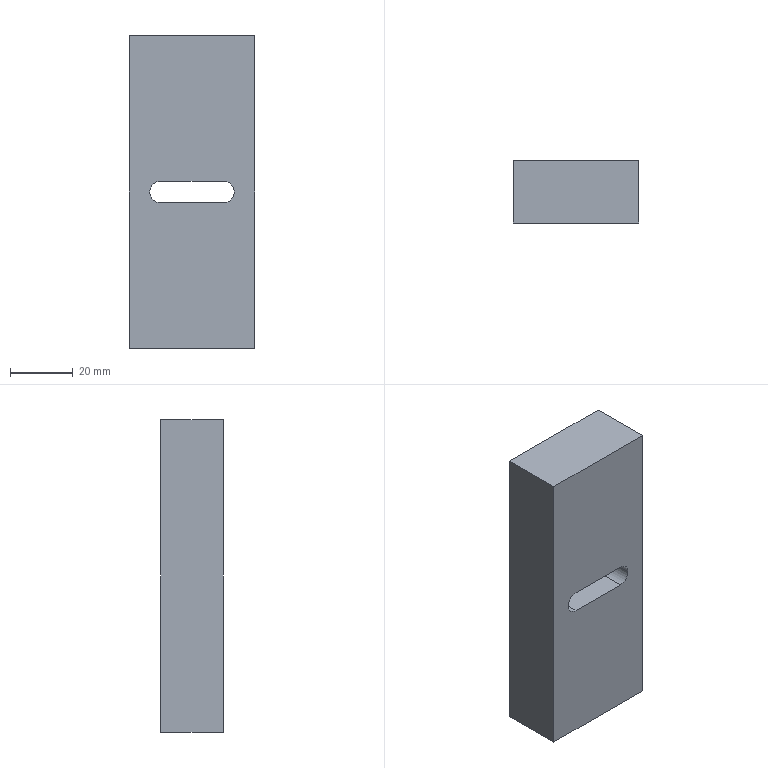Component | SolidWorks | GuidePlate1-4 | 1 solid | 11 faces | box 40 x 20 x 100 mm | volume 76430 mm3 | plane 8 | cylinder 3 | commonest cylinder face diameters 7 x3
build123d program:
from build123d import *

# Parameters (mm, degrees)
SKETCH1_W           = 40
SKETCH1_H           = 100
BOSS_EXTRUDE1_DEPTH = 20
CUT_EXTRUDE1_DEPTH  = 110.545


with BuildPart() as part:
    # Sketch1 → Boss-Extrude1 (new body)
    with BuildSketch(Plane.XY):
        with Locations((20, -50)):
            Rectangle(SKETCH1_W, SKETCH1_H)
    extrude(amount=BOSS_EXTRUDE1_DEPTH)

    # Sketch2 → Cut-Extrude1 (cut, through all)
    with BuildSketch(Plane(origin=(0, 0, 0), x_dir=(-1, 0, 0), z_dir=(0, 0, -1))):
        with BuildLine():
            Line((-30, -46.5), (-10, -46.5))
            ThreePointArc((-10, -46.5), (-6.5, -50), (-10, -53.5))
            Line((-10, -53.5), (-30, -53.5))
            ThreePointArc((-30, -53.5), (-33.5, -50), (-30, -46.5))
        make_face()
    extrude(amount=-CUT_EXTRUDE1_DEPTH, mode=Mode.SUBTRACT)


solid = part.part

# Placed as in the assembly
solid = solid.moved(Location((-367.951, 457.323, -225), (90, 0, 0)))
STEP:
#1=CARTESIAN_POINT('',(-13.167,18.005,-10.827));
#2=VERTEX_POINT('',#1);
#3=CARTESIAN_POINT('',(-13.305,18.005,-10.689));
#4=VERTEX_POINT('',#3);
#5=CARTESIAN_POINT('',(-13.305,18.005,-10.827));
#6=DIRECTION('',(-0.,-1.,-0.));
#7=DIRECTION('',(1.,0.,0.));
#8=AXIS2_PLACEMENT_3D('',#5,#6,#7);
#9=CIRCLE('',#8,0.1378);
#10=EDGE_CURVE('',#2,#4,#9,.T.);
#11=ORIENTED_EDGE('',*,*,#10,.F.);
#12=CARTESIAN_POINT('',(-13.167,17.217,-10.827));
#13=VERTEX_POINT('',#12);
#14=CARTESIAN_POINT('',(-13.167,18.005,-10.827));
#15=DIRECTION('',(-0.,-1.,-0.));
#16=VECTOR('',#15,39.37);
#17=LINE('',#14,#16);
#18=EDGE_CURVE('',#2,#13,#17,.T.);
#19=ORIENTED_EDGE('',*,*,#18,.T.);
#20=CARTESIAN_POINT('',(-13.305,17.217,-10.689));
#21=VERTEX_POINT('',#20);
#22=CARTESIAN_POINT('',(-13.305,17.217,-10.827));
#23=DIRECTION('',(-0.,-1.,-0.));
#24=DIRECTION('',(1.,0.,0.));
#25=AXIS2_PLACEMENT_3D('',#22,#23,#24);
#26=CIRCLE('',#25,0.1378);
#27=EDGE_CURVE('',#13,#21,#26,.T.);
#28=ORIENTED_EDGE('',*,*,#27,.T.);
#29=CARTESIAN_POINT('',(-13.305,18.005,-10.689));
#30=DIRECTION('',(-0.,-1.,-0.));
#31=VECTOR('',#30,39.37);
#32=LINE('',#29,#31);
#33=EDGE_CURVE('',#4,#21,#32,.T.);
#34=ORIENTED_EDGE('',*,*,#33,.F.);
#35=EDGE_LOOP('',(#11,#19,#28,#34));
#36=FACE_OUTER_BOUND('',#35,.T.);
#37=CARTESIAN_POINT('',(-13.305,18.005,-10.827));
#38=DIRECTION('',(-0.,-1.,-0.));
#39=DIRECTION('',(1.,0.,0.));
#40=AXIS2_PLACEMENT_3D('',#37,#38,#39);
#41=CYLINDRICAL_SURFACE('',#40,0.1378);
#42=ADVANCED_FACE('',(#36),#41,.F.);
#43=CARTESIAN_POINT('',(-12.911,17.217,-8.858));
#44=VERTEX_POINT('',#43);
#45=CARTESIAN_POINT('',(-12.911,17.217,-12.795));
#46=VERTEX_POINT('',#45);
#47=CARTESIAN_POINT('',(-12.911,17.217,-8.858));
#48=DIRECTION('',(-0.,0.,-1.));
#49=VECTOR('',#48,39.37);
#50=LINE('',#47,#49);
#51=EDGE_CURVE('',#44,#46,#50,.T.);
#52=ORIENTED_EDGE('',*,*,#51,.T.);
#53=CARTESIAN_POINT('',(-12.911,18.005,-12.795));
#54=VERTEX_POINT('',#53);
#55=CARTESIAN_POINT('',(-12.911,18.005,-12.795));
#56=DIRECTION('',(-0.,-1.,-0.));
#57=VECTOR('',#56,39.37);
#58=LINE('',#55,#57);
#59=EDGE_CURVE('',#54,#46,#58,.T.);
#60=ORIENTED_EDGE('',*,*,#59,.F.);
#61=CARTESIAN_POINT('',(-12.911,18.005,-8.858));
#62=VERTEX_POINT('',#61);
#63=CARTESIAN_POINT('',(-12.911,18.005,-8.858));
#64=DIRECTION('',(-0.,0.,-1.));
#65=VECTOR('',#64,39.37);
#66=LINE('',#63,#65);
#67=EDGE_CURVE('',#62,#54,#66,.T.);
#68=ORIENTED_EDGE('',*,*,#67,.F.);
#69=CARTESIAN_POINT('',(-12.911,18.005,-8.858));
#70=DIRECTION('',(-0.,-1.,-0.));
#71=VECTOR('',#70,39.37);
#72=LINE('',#69,#71);
#73=EDGE_CURVE('',#62,#44,#72,.T.);
#74=ORIENTED_EDGE('',*,*,#73,.T.);
#75=EDGE_LOOP('',(#52,#60,#68,#74));
#76=FACE_OUTER_BOUND('',#75,.T.);
#77=CARTESIAN_POINT('',(-12.911,18.005,-8.858));
#78=DIRECTION('',(-1.,0.,0.));
#79=DIRECTION('',(0.,-0.,1.));
#80=AXIS2_PLACEMENT_3D('',#77,#78,#79);
#81=PLANE('',#80);
#82=ADVANCED_FACE('',(#76),#81,.F.);
#83=CARTESIAN_POINT('',(-14.486,17.217,-12.795));
#84=VERTEX_POINT('',#83);
#85=CARTESIAN_POINT('',(-12.911,17.217,-12.795));
#86=DIRECTION('',(-1.,0.,0.));
#87=VECTOR('',#86,39.37);
#88=LINE('',#85,#87);
#89=EDGE_CURVE('',#46,#84,#88,.T.);
#90=ORIENTED_EDGE('',*,*,#89,.T.);
#91=CARTESIAN_POINT('',(-14.486,18.005,-12.795));
#92=VERTEX_POINT('',#91);
#93=CARTESIAN_POINT('',(-14.486,18.005,-12.795));
#94=DIRECTION('',(-0.,-1.,-0.));
#95=VECTOR('',#94,39.37);
#96=LINE('',#93,#95);
#97=EDGE_CURVE('',#92,#84,#96,.T.);
#98=ORIENTED_EDGE('',*,*,#97,.F.);
#99=CARTESIAN_POINT('',(-12.911,18.005,-12.795));
#100=DIRECTION('',(-1.,0.,0.));
#101=VECTOR('',#100,39.37);
#102=LINE('',#99,#101);
#103=EDGE_CURVE('',#54,#92,#102,.T.);
#104=ORIENTED_EDGE('',*,*,#103,.F.);
#105=ORIENTED_EDGE('',*,*,#59,.T.);
#106=EDGE_LOOP('',(#90,#98,#104,#105));
#107=FACE_OUTER_BOUND('',#106,.T.);
#108=CARTESIAN_POINT('',(-12.911,18.005,-12.795));
#109=DIRECTION('',(0.,-0.,1.));
#110=DIRECTION('',(0.,1.,0.));
#111=AXIS2_PLACEMENT_3D('',#108,#109,#110);
#112=PLANE('',#111);
#113=ADVANCED_FACE('',(#107),#112,.F.);
#114=CARTESIAN_POINT('',(-14.486,17.217,-8.858));
#115=VERTEX_POINT('',#114);
#116=CARTESIAN_POINT('',(-14.486,17.217,-8.858));
#117=DIRECTION('',(0.,-0.,1.));
#118=VECTOR('',#117,39.37);
#119=LINE('',#116,#118);
#120=EDGE_CURVE('',#84,#115,#119,.T.);
#121=ORIENTED_EDGE('',*,*,#120,.T.);
#122=CARTESIAN_POINT('',(-14.486,18.005,-8.858));
#123=VERTEX_POINT('',#122);
#124=CARTESIAN_POINT('',(-14.486,18.005,-8.858));
#125=DIRECTION('',(-0.,-1.,-0.));
#126=VECTOR('',#125,39.37);
#127=LINE('',#124,#126);
#128=EDGE_CURVE('',#123,#115,#127,.T.);
#129=ORIENTED_EDGE('',*,*,#128,.F.);
#130=CARTESIAN_POINT('',(-14.486,18.005,-8.858));
#131=DIRECTION('',(0.,-0.,1.));
#132=VECTOR('',#131,39.37);
#133=LINE('',#130,#132);
#134=EDGE_CURVE('',#92,#123,#133,.T.);
#135=ORIENTED_EDGE('',*,*,#134,.F.);
#136=ORIENTED_EDGE('',*,*,#97,.T.);
#137=EDGE_LOOP('',(#121,#129,#135,#136));
#138=FACE_OUTER_BOUND('',#137,.T.);
#139=CARTESIAN_POINT('',(-14.486,18.005,-8.858));
#140=DIRECTION('',(1.,-0.,-0.));
#141=DIRECTION('',(-0.,0.,-1.));
#142=AXIS2_PLACEMENT_3D('',#139,#140,#141);
#143=PLANE('',#142);
#144=ADVANCED_FACE('',(#138),#143,.F.);
#145=CARTESIAN_POINT('',(-12.911,17.217,-8.858));
#146=DIRECTION('',(1.,-0.,-0.));
#147=VECTOR('',#146,39.37);
#148=LINE('',#145,#147);
#149=EDGE_CURVE('',#115,#44,#148,.T.);
#150=ORIENTED_EDGE('',*,*,#149,.T.);
#151=ORIENTED_EDGE('',*,*,#73,.F.);
#152=CARTESIAN_POINT('',(-12.911,18.005,-8.858));
#153=DIRECTION('',(1.,-0.,-0.));
#154=VECTOR('',#153,39.37);
#155=LINE('',#152,#154);
#156=EDGE_CURVE('',#123,#62,#155,.T.);
#157=ORIENTED_EDGE('',*,*,#156,.F.);
#158=ORIENTED_EDGE('',*,*,#128,.T.);
#159=EDGE_LOOP('',(#150,#151,#157,#158));
#160=FACE_OUTER_BOUND('',#159,.T.);
#161=CARTESIAN_POINT('',(-12.911,18.005,-8.858));
#162=DIRECTION('',(-0.,0.,-1.));
#163=DIRECTION('',(-0.,-1.,-0.));
#164=AXIS2_PLACEMENT_3D('',#161,#162,#163);
#165=PLANE('',#164);
#166=ADVANCED_FACE('',(#160),#165,.F.);
#167=CARTESIAN_POINT('',(-14.093,18.005,-10.689));
#168=VERTEX_POINT('',#167);
#169=CARTESIAN_POINT('',(-14.093,18.005,-10.965));
#170=VERTEX_POINT('',#169);
#171=CARTESIAN_POINT('',(-14.093,18.005,-10.827));
#172=DIRECTION('',(-0.,-1.,-0.));
#173=DIRECTION('',(1.,0.,0.));
#174=AXIS2_PLACEMENT_3D('',#171,#172,#173);
#175=CIRCLE('',#174,0.1378);
#176=EDGE_CURVE('',#168,#170,#175,.T.);
#177=ORIENTED_EDGE('',*,*,#176,.T.);
#178=CARTESIAN_POINT('',(-13.305,18.005,-10.965));
#179=VERTEX_POINT('',#178);
#180=CARTESIAN_POINT('',(-14.093,18.005,-10.965));
#181=DIRECTION('',(1.,-0.,-0.));
#182=VECTOR('',#181,39.37);
#183=LINE('',#180,#182);
#184=EDGE_CURVE('',#170,#179,#183,.T.);
#185=ORIENTED_EDGE('',*,*,#184,.T.);
#186=CARTESIAN_POINT('',(-13.305,18.005,-10.827));
#187=DIRECTION('',(-0.,-1.,-0.));
#188=DIRECTION('',(1.,0.,0.));
#189=AXIS2_PLACEMENT_3D('',#186,#187,#188);
#190=CIRCLE('',#189,0.1378);
#191=EDGE_CURVE('',#179,#2,#190,.T.);
#192=ORIENTED_EDGE('',*,*,#191,.T.);
#193=ORIENTED_EDGE('',*,*,#10,.T.);
#194=CARTESIAN_POINT('',(-14.093,18.005,-10.689));
#195=DIRECTION('',(-1.,0.,0.));
#196=VECTOR('',#195,39.37);
#197=LINE('',#194,#196);
#198=EDGE_CURVE('',#4,#168,#197,.T.);
#199=ORIENTED_EDGE('',*,*,#198,.T.);
#200=EDGE_LOOP('',(#177,#185,#192,#193,#199));
#201=FACE_BOUND('',#200,.T.);
#202=ORIENTED_EDGE('',*,*,#67,.T.);
#203=ORIENTED_EDGE('',*,*,#103,.T.);
#204=ORIENTED_EDGE('',*,*,#134,.T.);
#205=ORIENTED_EDGE('',*,*,#156,.T.);
#206=EDGE_LOOP('',(#202,#203,#204,#205));
#207=FACE_OUTER_BOUND('',#206,.T.);
#208=CARTESIAN_POINT('',(-12.911,18.005,-8.858));
#209=DIRECTION('',(0.,1.,0.));
#210=DIRECTION('',(-1.,0.,0.));
#211=AXIS2_PLACEMENT_3D('',#208,#209,#210);
#212=PLANE('',#211);
#213=ADVANCED_FACE('',(#201,#207),#212,.T.);
#214=CARTESIAN_POINT('',(-14.093,17.217,-10.965));
#215=VERTEX_POINT('',#214);
#216=CARTESIAN_POINT('',(-13.305,17.217,-10.965));
#217=VERTEX_POINT('',#216);
#218=CARTESIAN_POINT('',(-14.093,17.217,-10.965));
#219=DIRECTION('',(1.,-0.,-0.));
#220=VECTOR('',#219,39.37);
#221=LINE('',#218,#220);
#222=EDGE_CURVE('',#215,#217,#221,.T.);
#223=ORIENTED_EDGE('',*,*,#222,.F.);
#224=CARTESIAN_POINT('',(-14.093,17.217,-10.689));
#225=VERTEX_POINT('',#224);
#226=CARTESIAN_POINT('',(-14.093,17.217,-10.827));
#227=DIRECTION('',(-0.,-1.,-0.));
#228=DIRECTION('',(1.,0.,0.));
#229=AXIS2_PLACEMENT_3D('',#226,#227,#228);
#230=CIRCLE('',#229,0.1378);
#231=EDGE_CURVE('',#225,#215,#230,.T.);
#232=ORIENTED_EDGE('',*,*,#231,.F.);
#233=CARTESIAN_POINT('',(-14.093,17.217,-10.689));
#234=DIRECTION('',(-1.,0.,0.));
#235=VECTOR('',#234,39.37);
#236=LINE('',#233,#235);
#237=EDGE_CURVE('',#21,#225,#236,.T.);
#238=ORIENTED_EDGE('',*,*,#237,.F.);
#239=ORIENTED_EDGE('',*,*,#27,.F.);
#240=CARTESIAN_POINT('',(-13.305,17.217,-10.827));
#241=DIRECTION('',(-0.,-1.,-0.));
#242=DIRECTION('',(1.,0.,0.));
#243=AXIS2_PLACEMENT_3D('',#240,#241,#242);
#244=CIRCLE('',#243,0.1378);
#245=EDGE_CURVE('',#217,#13,#244,.T.);
#246=ORIENTED_EDGE('',*,*,#245,.F.);
#247=EDGE_LOOP('',(#223,#232,#238,#239,#246));
#248=FACE_BOUND('',#247,.T.);
#249=ORIENTED_EDGE('',*,*,#51,.F.);
#250=ORIENTED_EDGE('',*,*,#149,.F.);
#251=ORIENTED_EDGE('',*,*,#120,.F.);
#252=ORIENTED_EDGE('',*,*,#89,.F.);
#253=EDGE_LOOP('',(#249,#250,#251,#252));
#254=FACE_OUTER_BOUND('',#253,.T.);
#255=CARTESIAN_POINT('',(-12.911,17.217,-8.858));
#256=DIRECTION('',(0.,1.,0.));
#257=DIRECTION('',(-1.,0.,0.));
#258=AXIS2_PLACEMENT_3D('',#255,#256,#257);
#259=PLANE('',#258);
#260=ADVANCED_FACE('',(#248,#254),#259,.F.);
#261=ORIENTED_EDGE('',*,*,#231,.T.);
#262=CARTESIAN_POINT('',(-14.093,18.005,-10.965));
#263=DIRECTION('',(-0.,-1.,-0.));
#264=VECTOR('',#263,39.37);
#265=LINE('',#262,#264);
#266=EDGE_CURVE('',#170,#215,#265,.T.);
#267=ORIENTED_EDGE('',*,*,#266,.F.);
#268=ORIENTED_EDGE('',*,*,#176,.F.);
#269=CARTESIAN_POINT('',(-14.093,18.005,-10.689));
#270=DIRECTION('',(-0.,-1.,-0.));
#271=VECTOR('',#270,39.37);
#272=LINE('',#269,#271);
#273=EDGE_CURVE('',#168,#225,#272,.T.);
#274=ORIENTED_EDGE('',*,*,#273,.T.);
#275=EDGE_LOOP('',(#261,#267,#268,#274));
#276=FACE_OUTER_BOUND('',#275,.T.);
#277=CARTESIAN_POINT('',(-14.093,18.005,-10.827));
#278=DIRECTION('',(-0.,-1.,-0.));
#279=DIRECTION('',(1.,0.,0.));
#280=AXIS2_PLACEMENT_3D('',#277,#278,#279);
#281=CYLINDRICAL_SURFACE('',#280,0.1378);
#282=ADVANCED_FACE('',(#276),#281,.F.);
#283=ORIENTED_EDGE('',*,*,#237,.T.);
#284=ORIENTED_EDGE('',*,*,#273,.F.);
#285=ORIENTED_EDGE('',*,*,#198,.F.);
#286=ORIENTED_EDGE('',*,*,#33,.T.);
#287=EDGE_LOOP('',(#283,#284,#285,#286));
#288=FACE_OUTER_BOUND('',#287,.T.);
#289=CARTESIAN_POINT('',(-14.093,18.005,-10.689));
#290=DIRECTION('',(0.,-0.,1.));
#291=DIRECTION('',(0.,1.,0.));
#292=AXIS2_PLACEMENT_3D('',#289,#290,#291);
#293=PLANE('',#292);
#294=ADVANCED_FACE('',(#288),#293,.F.);
#295=ORIENTED_EDGE('',*,*,#18,.F.);
#296=ORIENTED_EDGE('',*,*,#191,.F.);
#297=CARTESIAN_POINT('',(-13.305,18.005,-10.965));
#298=DIRECTION('',(-0.,-1.,-0.));
#299=VECTOR('',#298,39.37);
#300=LINE('',#297,#299);
#301=EDGE_CURVE('',#179,#217,#300,.T.);
#302=ORIENTED_EDGE('',*,*,#301,.T.);
#303=ORIENTED_EDGE('',*,*,#245,.T.);
#304=EDGE_LOOP('',(#295,#296,#302,#303));
#305=FACE_OUTER_BOUND('',#304,.T.);
#306=CARTESIAN_POINT('',(-13.305,18.005,-10.827));
#307=DIRECTION('',(-0.,-1.,-0.));
#308=DIRECTION('',(1.,0.,0.));
#309=AXIS2_PLACEMENT_3D('',#306,#307,#308);
#310=CYLINDRICAL_SURFACE('',#309,0.1378);
#311=ADVANCED_FACE('',(#305),#310,.F.);
#312=ORIENTED_EDGE('',*,*,#222,.T.);
#313=ORIENTED_EDGE('',*,*,#301,.F.);
#314=ORIENTED_EDGE('',*,*,#184,.F.);
#315=ORIENTED_EDGE('',*,*,#266,.T.);
#316=EDGE_LOOP('',(#312,#313,#314,#315));
#317=FACE_OUTER_BOUND('',#316,.T.);
#318=CARTESIAN_POINT('',(-14.093,18.005,-10.965));
#319=DIRECTION('',(-0.,0.,-1.));
#320=DIRECTION('',(-0.,-1.,-0.));
#321=AXIS2_PLACEMENT_3D('',#318,#319,#320);
#322=PLANE('',#321);
#323=ADVANCED_FACE('',(#317),#322,.F.);
#324=CLOSED_SHELL('',(#42,#82,#113,#144,#166,#213,#260,#282,#294,#311,#323));
#325=MANIFOLD_SOLID_BREP('',#324);
#326=CARTESIAN_POINT('',(0.,0.,0.));
#327=DIRECTION('',(0.,0.,1.));
#328=DIRECTION('',(1.,0.,0.));
#329=AXIS2_PLACEMENT_3D('',#326,#327,#328);
#330=(LENGTH_UNIT()NAMED_UNIT(*)SI_UNIT($,.METRE.));
#331=LENGTH_MEASURE_WITH_UNIT(LENGTH_MEASURE(0.0254),#330);
#332=DIMENSIONAL_EXPONENTS(1.,0.,0.,0.,0.,0.,0.);
#333=(CONVERSION_BASED_UNIT('',#331)LENGTH_UNIT()NAMED_UNIT(#332));
#334=UNCERTAINTY_MEASURE_WITH_UNIT(LENGTH_MEASURE(0.00001),#333,'','');
#335=(NAMED_UNIT(*)PLANE_ANGLE_UNIT()SI_UNIT($,.RADIAN.));
#336=(NAMED_UNIT(*)SI_UNIT($,.STERADIAN.)SOLID_ANGLE_UNIT());
#337=(GEOMETRIC_REPRESENTATION_CONTEXT(3)GLOBAL_UNCERTAINTY_ASSIGNED_CONTEXT((#334))GLOBAL_UNIT_ASSIGNED_CONTEXT((#333,#335,#336))REPRESENTATION_CONTEXT('',''));
#338=ADVANCED_BREP_SHAPE_REPRESENTATION('',(#325,#329),#337);
#339=COLOUR_RGB('',0.7922,0.8196,0.9333);
#340=FILL_AREA_STYLE_COLOUR('',#339);
#341=FILL_AREA_STYLE('',(#340));
#342=SURFACE_STYLE_FILL_AREA(#341);
#343=SURFACE_SIDE_STYLE('',(#342));
#344=SURFACE_STYLE_USAGE(.BOTH.,#343);
#345=PRESENTATION_STYLE_ASSIGNMENT((#344));
#346=STYLED_ITEM('',(#345),#325);
#347=(LENGTH_UNIT()NAMED_UNIT(*)SI_UNIT($,.METRE.));
#348=LENGTH_MEASURE_WITH_UNIT(LENGTH_MEASURE(0.0254),#347);
#349=DIMENSIONAL_EXPONENTS(1.,0.,0.,0.,0.,0.,0.);
#350=(CONVERSION_BASED_UNIT('',#348)LENGTH_UNIT()NAMED_UNIT(#349));
#351=UNCERTAINTY_MEASURE_WITH_UNIT(LENGTH_MEASURE(0.00001),#350,'','');
#352=(NAMED_UNIT(*)PLANE_ANGLE_UNIT()SI_UNIT($,.RADIAN.));
#353=(NAMED_UNIT(*)SI_UNIT($,.STERADIAN.)SOLID_ANGLE_UNIT());
#354=(GEOMETRIC_REPRESENTATION_CONTEXT(3)GLOBAL_UNCERTAINTY_ASSIGNED_CONTEXT((#351))GLOBAL_UNIT_ASSIGNED_CONTEXT((#350,#352,#353))REPRESENTATION_CONTEXT('',''));
#355=MECHANICAL_DESIGN_GEOMETRIC_PRESENTATION_REPRESENTATION('',(#346),#354);
#356=PRESENTATION_LAYER_ASSIGNMENT('','',(#346));